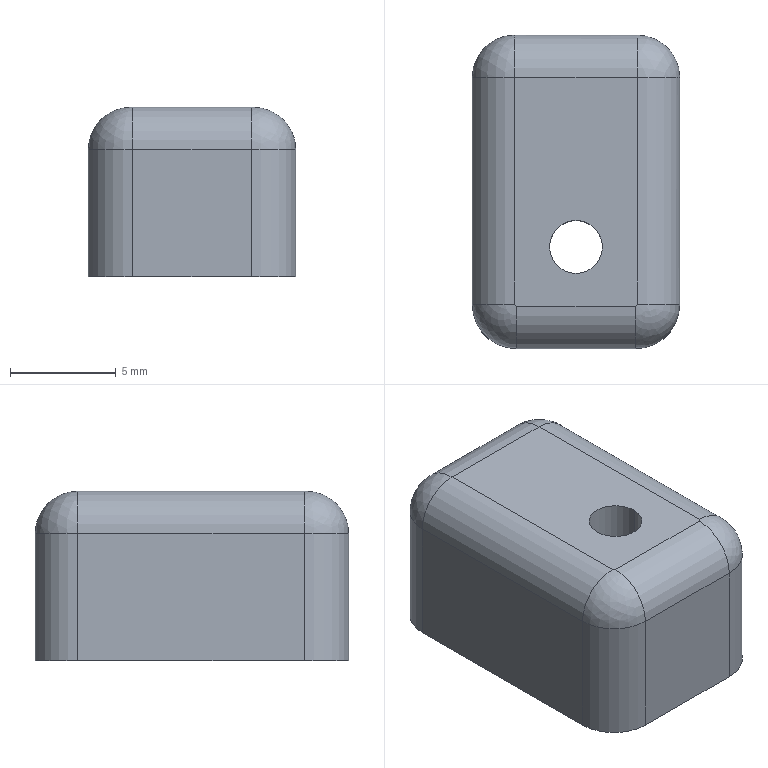CAM job | Mastercam | mm | 2 operations | part box 9.8 x 14.8 x 8
1. Unified Morph | 5 - 4 圆鼻铣刀
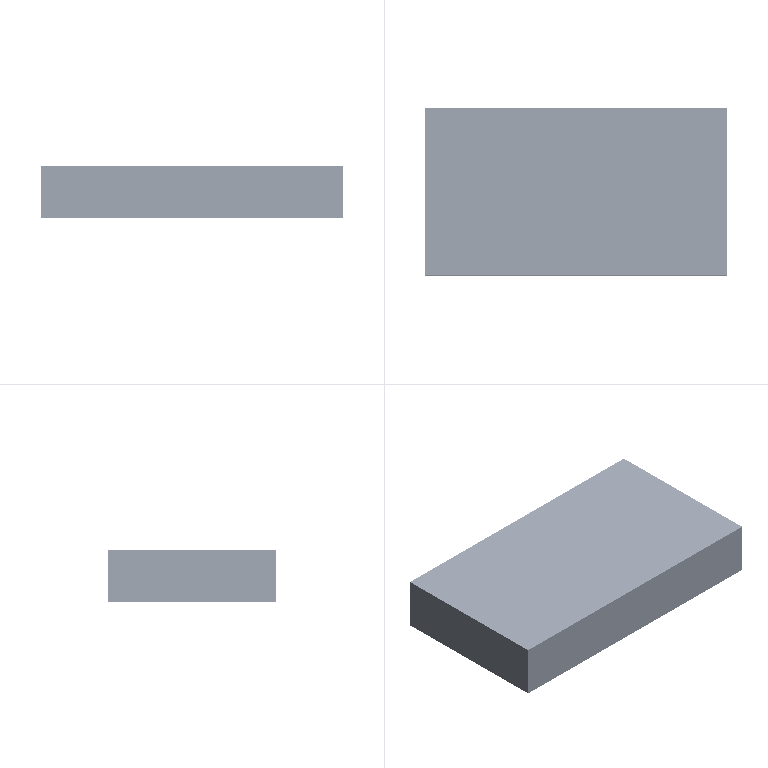2. Surface Finish Flowline | 5 - 4 圆鼻铣刀